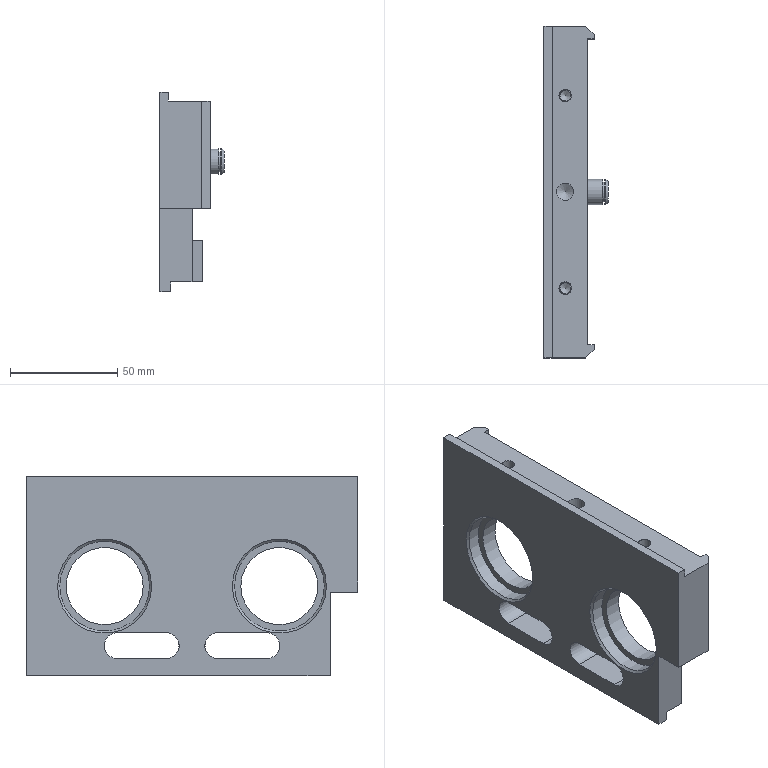Component | NX | RIGHT_SIDE_PLATE | 1 solid | 76 faces | volume 160131 mm3 | plane 38 | cylinder 25 | cone 13 | commonest cylinder face diameters 12 x6 5.795 x4 5 x4 36 x2 20 x2 8 x2 42 x2 16 x1